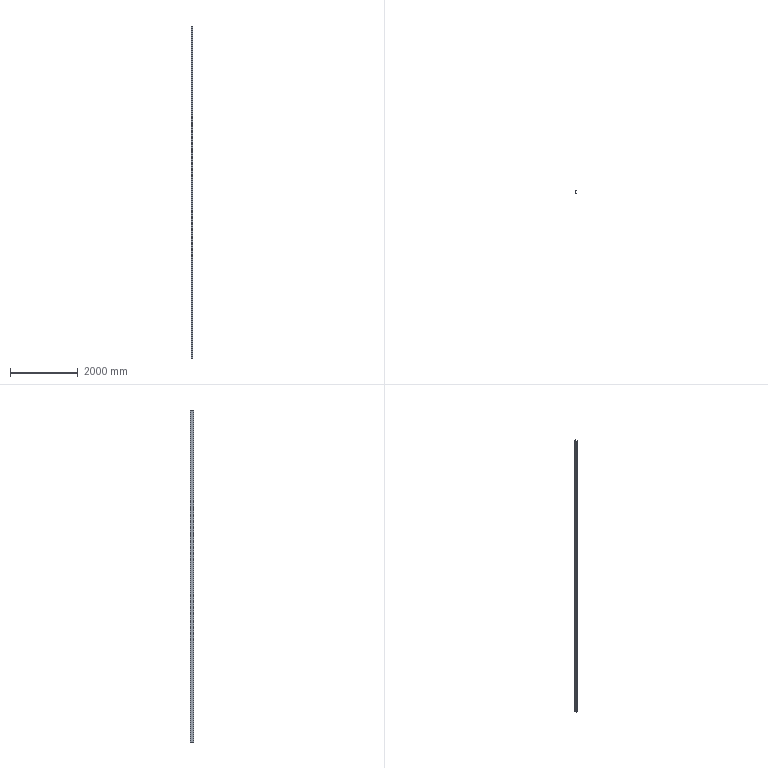Component | NX | CHUNSHUIJINCAO_CAOGANG | 1 solid | 10 faces | box 48 x 100 x 9820 mm | volume 12332938 mm3 | plane 10
STEP:
#1=CARTESIAN_POINT('',(0.,0.,0.));
#2=DIRECTION('',(0.,0.,1.));
#3=DIRECTION('',(1.,0.,0.));
#4=AXIS2_PLACEMENT_3D('',#1,#2,#3);
#5=CARTESIAN_POINT('',(2050.,9250.,9960.));
#6=VERTEX_POINT('',#5);
#7=CARTESIAN_POINT('',(2098.,9250.,9960.));
#8=VERTEX_POINT('',#7);
#9=CARTESIAN_POINT('',(2050.,9250.,9960.));
#10=DIRECTION('',(1.,0.,0.));
#11=VECTOR('',#10,1.);
#12=LINE('',#9,#11);
#13=CARTESIAN_POINT('',(2050.,9250.,140.));
#14=DIRECTION('',(0.,-1.,0.));
#15=DIRECTION('',(-1.,-0.,0.));
#16=AXIS2_PLACEMENT_3D('',#13,#14,#15);
#17=PLANE('',#16);
#18=CARTESIAN_POINT('',(0.,-9820.));
#19=DIRECTION('',(-1.,0.));
#20=VECTOR('',#19,1.);
#21=LINE('',#18,#20);
#22=(GEOMETRIC_REPRESENTATION_CONTEXT(2)PARAMETRIC_REPRESENTATION_CONTEXT()REPRESENTATION_CONTEXT('',''));
#23=DEFINITIONAL_REPRESENTATION('',(#21),#22);
#24=PCURVE('',#17,#23);
#25=CARTESIAN_POINT('',(2050.,9250.,9960.));
#26=DIRECTION('',(0.,0.,1.));
#27=DIRECTION('',(0.,-1.,0.));
#28=AXIS2_PLACEMENT_3D('',#25,#26,#27);
#29=PLANE('',#28);
#30=CARTESIAN_POINT('',(0.,0.));
#31=DIRECTION('',(-0.,1.));
#32=VECTOR('',#31,1.);
#33=LINE('',#30,#32);
#34=(GEOMETRIC_REPRESENTATION_CONTEXT(2)PARAMETRIC_REPRESENTATION_CONTEXT()REPRESENTATION_CONTEXT('',''));
#35=DEFINITIONAL_REPRESENTATION('',(#33),#34);
#36=PCURVE('',#29,#35);
#37=SURFACE_CURVE('',#12,(#24,#36),.PCURVE_S1.);
#38=EDGE_CURVE('',#6,#8,#37,.T.);
#39=ORIENTED_EDGE('',*,*,#38,.F.);
#40=CARTESIAN_POINT('',(2050.,9250.,140.));
#41=VERTEX_POINT('',#40);
#42=CARTESIAN_POINT('',(2050.,9250.,140.));
#43=DIRECTION('',(0.,0.,1.));
#44=VECTOR('',#43,1.);
#45=LINE('',#42,#44);
#46=CARTESIAN_POINT('',(0.,0.));
#47=DIRECTION('',(0.,-1.));
#48=VECTOR('',#47,1.);
#49=LINE('',#46,#48);
#50=(GEOMETRIC_REPRESENTATION_CONTEXT(2)PARAMETRIC_REPRESENTATION_CONTEXT()REPRESENTATION_CONTEXT('',''));
#51=DEFINITIONAL_REPRESENTATION('',(#49),#50);
#52=PCURVE('',#17,#51);
#53=CARTESIAN_POINT('',(2050.,9350.,140.));
#54=DIRECTION('',(-1.,0.,0.));
#55=DIRECTION('',(0.,0.,1.));
#56=AXIS2_PLACEMENT_3D('',#53,#54,#55);
#57=PLANE('',#56);
#58=CARTESIAN_POINT('',(0.,-100.));
#59=DIRECTION('',(1.,0.));
#60=VECTOR('',#59,1.);
#61=LINE('',#58,#60);
#62=(GEOMETRIC_REPRESENTATION_CONTEXT(2)PARAMETRIC_REPRESENTATION_CONTEXT()REPRESENTATION_CONTEXT('',''));
#63=DEFINITIONAL_REPRESENTATION('',(#61),#62);
#64=PCURVE('',#57,#63);
#65=SURFACE_CURVE('',#45,(#52,#64),.PCURVE_S1.);
#66=EDGE_CURVE('',#41,#6,#65,.T.);
#67=ORIENTED_EDGE('',*,*,#66,.F.);
#68=CARTESIAN_POINT('',(2098.,9250.,140.));
#69=VERTEX_POINT('',#68);
#70=CARTESIAN_POINT('',(2050.,9250.,140.));
#71=DIRECTION('',(1.,0.,0.));
#72=VECTOR('',#71,1.);
#73=LINE('',#70,#72);
#74=CARTESIAN_POINT('',(0.,0.));
#75=DIRECTION('',(-1.,0.));
#76=VECTOR('',#75,1.);
#77=LINE('',#74,#76);
#78=(GEOMETRIC_REPRESENTATION_CONTEXT(2)PARAMETRIC_REPRESENTATION_CONTEXT()REPRESENTATION_CONTEXT('',''));
#79=DEFINITIONAL_REPRESENTATION('',(#77),#78);
#80=PCURVE('',#17,#79);
#81=CARTESIAN_POINT('',(2050.,9250.,140.));
#82=DIRECTION('',(0.,0.,1.));
#83=DIRECTION('',(0.,-1.,0.));
#84=AXIS2_PLACEMENT_3D('',#81,#82,#83);
#85=PLANE('',#84);
#86=CARTESIAN_POINT('',(0.,0.));
#87=DIRECTION('',(-0.,1.));
#88=VECTOR('',#87,1.);
#89=LINE('',#86,#88);
#90=(GEOMETRIC_REPRESENTATION_CONTEXT(2)PARAMETRIC_REPRESENTATION_CONTEXT()REPRESENTATION_CONTEXT('',''));
#91=DEFINITIONAL_REPRESENTATION('',(#89),#90);
#92=PCURVE('',#85,#91);
#93=SURFACE_CURVE('',#73,(#80,#92),.PCURVE_S1.);
#94=EDGE_CURVE('',#41,#69,#93,.T.);
#95=ORIENTED_EDGE('',*,*,#94,.T.);
#96=CARTESIAN_POINT('',(2098.,9250.,140.));
#97=DIRECTION('',(0.,0.,1.));
#98=VECTOR('',#97,1.);
#99=LINE('',#96,#98);
#100=CARTESIAN_POINT('',(-48.,0.));
#101=DIRECTION('',(0.,-1.));
#102=VECTOR('',#101,1.);
#103=LINE('',#100,#102);
#104=(GEOMETRIC_REPRESENTATION_CONTEXT(2)PARAMETRIC_REPRESENTATION_CONTEXT()REPRESENTATION_CONTEXT('',''));
#105=DEFINITIONAL_REPRESENTATION('',(#103),#104);
#106=PCURVE('',#17,#105);
#107=CARTESIAN_POINT('',(2098.,9250.,140.));
#108=DIRECTION('',(1.,0.,0.));
#109=DIRECTION('',(0.,0.,-1.));
#110=AXIS2_PLACEMENT_3D('',#107,#108,#109);
#111=PLANE('',#110);
#112=CARTESIAN_POINT('',(0.,0.));
#113=DIRECTION('',(-1.,0.));
#114=VECTOR('',#113,1.);
#115=LINE('',#112,#114);
#116=(GEOMETRIC_REPRESENTATION_CONTEXT(2)PARAMETRIC_REPRESENTATION_CONTEXT()REPRESENTATION_CONTEXT('',''));
#117=DEFINITIONAL_REPRESENTATION('',(#115),#116);
#118=PCURVE('',#111,#117);
#119=SURFACE_CURVE('',#99,(#106,#118),.PCURVE_S1.);
#120=EDGE_CURVE('',#69,#8,#119,.T.);
#121=ORIENTED_EDGE('',*,*,#120,.T.);
#122=EDGE_LOOP('',(#39,#67,#95,#121));
#123=FACE_BOUND('',#122,.T.);
#124=ADVANCED_FACE('',(#123),#17,.T.);
#125=CARTESIAN_POINT('',(2098.,9258.5,9960.));
#126=VERTEX_POINT('',#125);
#127=CARTESIAN_POINT('',(2098.,9250.,9960.));
#128=DIRECTION('',(0.,1.,0.));
#129=VECTOR('',#128,1.);
#130=LINE('',#127,#129);
#131=CARTESIAN_POINT('',(-9820.,0.));
#132=DIRECTION('',(0.,1.));
#133=VECTOR('',#132,1.);
#134=LINE('',#131,#133);
#135=(GEOMETRIC_REPRESENTATION_CONTEXT(2)PARAMETRIC_REPRESENTATION_CONTEXT()REPRESENTATION_CONTEXT('',''));
#136=DEFINITIONAL_REPRESENTATION('',(#134),#135);
#137=PCURVE('',#111,#136);
#138=CARTESIAN_POINT('',(0.,48.));
#139=DIRECTION('',(-1.,0.));
#140=VECTOR('',#139,1.);
#141=LINE('',#138,#140);
#142=(GEOMETRIC_REPRESENTATION_CONTEXT(2)PARAMETRIC_REPRESENTATION_CONTEXT()REPRESENTATION_CONTEXT('',''));
#143=DEFINITIONAL_REPRESENTATION('',(#141),#142);
#144=PCURVE('',#29,#143);
#145=SURFACE_CURVE('',#130,(#137,#144),.PCURVE_S1.);
#146=EDGE_CURVE('',#8,#126,#145,.T.);
#147=ORIENTED_EDGE('',*,*,#146,.F.);
#148=ORIENTED_EDGE('',*,*,#120,.F.);
#149=CARTESIAN_POINT('',(2098.,9258.5,140.));
#150=VERTEX_POINT('',#149);
#151=CARTESIAN_POINT('',(2098.,9250.,140.));
#152=DIRECTION('',(0.,1.,0.));
#153=VECTOR('',#152,1.);
#154=LINE('',#151,#153);
#155=CARTESIAN_POINT('',(0.,0.));
#156=DIRECTION('',(0.,1.));
#157=VECTOR('',#156,1.);
#158=LINE('',#155,#157);
#159=(GEOMETRIC_REPRESENTATION_CONTEXT(2)PARAMETRIC_REPRESENTATION_CONTEXT()REPRESENTATION_CONTEXT('',''));
#160=DEFINITIONAL_REPRESENTATION('',(#158),#159);
#161=PCURVE('',#111,#160);
#162=CARTESIAN_POINT('',(0.,48.));
#163=DIRECTION('',(-1.,0.));
#164=VECTOR('',#163,1.);
#165=LINE('',#162,#164);
#166=(GEOMETRIC_REPRESENTATION_CONTEXT(2)PARAMETRIC_REPRESENTATION_CONTEXT()REPRESENTATION_CONTEXT('',''));
#167=DEFINITIONAL_REPRESENTATION('',(#165),#166);
#168=PCURVE('',#85,#167);
#169=SURFACE_CURVE('',#154,(#161,#168),.PCURVE_S1.);
#170=EDGE_CURVE('',#69,#150,#169,.T.);
#171=ORIENTED_EDGE('',*,*,#170,.T.);
#172=CARTESIAN_POINT('',(2098.,9258.5,140.));
#173=DIRECTION('',(0.,0.,1.));
#174=VECTOR('',#173,1.);
#175=LINE('',#172,#174);
#176=CARTESIAN_POINT('',(0.,8.5));
#177=DIRECTION('',(-1.,0.));
#178=VECTOR('',#177,1.);
#179=LINE('',#176,#178);
#180=(GEOMETRIC_REPRESENTATION_CONTEXT(2)PARAMETRIC_REPRESENTATION_CONTEXT()REPRESENTATION_CONTEXT('',''));
#181=DEFINITIONAL_REPRESENTATION('',(#179),#180);
#182=PCURVE('',#111,#181);
#183=CARTESIAN_POINT('',(2098.,9258.5,140.));
#184=DIRECTION('',(-0.,1.,0.));
#185=DIRECTION('',(1.,0.,0.));
#186=AXIS2_PLACEMENT_3D('',#183,#184,#185);
#187=PLANE('',#186);
#188=CARTESIAN_POINT('',(0.,0.));
#189=DIRECTION('',(0.,-1.));
#190=VECTOR('',#189,1.);
#191=LINE('',#188,#190);
#192=(GEOMETRIC_REPRESENTATION_CONTEXT(2)PARAMETRIC_REPRESENTATION_CONTEXT()REPRESENTATION_CONTEXT('',''));
#193=DEFINITIONAL_REPRESENTATION('',(#191),#192);
#194=PCURVE('',#187,#193);
#195=SURFACE_CURVE('',#175,(#182,#194),.PCURVE_S1.);
#196=EDGE_CURVE('',#150,#126,#195,.T.);
#197=ORIENTED_EDGE('',*,*,#196,.T.);
#198=EDGE_LOOP('',(#147,#148,#171,#197));
#199=FACE_BOUND('',#198,.T.);
#200=ADVANCED_FACE('',(#199),#111,.T.);
#201=CARTESIAN_POINT('',(2055.3,9258.5,9960.));
#202=VERTEX_POINT('',#201);
#203=CARTESIAN_POINT('',(2098.,9258.5,9960.));
#204=DIRECTION('',(-1.,-0.,0.));
#205=VECTOR('',#204,1.);
#206=LINE('',#203,#205);
#207=CARTESIAN_POINT('',(0.,-9820.));
#208=DIRECTION('',(-1.,0.));
#209=VECTOR('',#208,1.);
#210=LINE('',#207,#209);
#211=(GEOMETRIC_REPRESENTATION_CONTEXT(2)PARAMETRIC_REPRESENTATION_CONTEXT()REPRESENTATION_CONTEXT('',''));
#212=DEFINITIONAL_REPRESENTATION('',(#210),#211);
#213=PCURVE('',#187,#212);
#214=CARTESIAN_POINT('',(-8.5,48.));
#215=DIRECTION('',(0.,-1.));
#216=VECTOR('',#215,1.);
#217=LINE('',#214,#216);
#218=(GEOMETRIC_REPRESENTATION_CONTEXT(2)PARAMETRIC_REPRESENTATION_CONTEXT()REPRESENTATION_CONTEXT('',''));
#219=DEFINITIONAL_REPRESENTATION('',(#217),#218);
#220=PCURVE('',#29,#219);
#221=SURFACE_CURVE('',#206,(#213,#220),.PCURVE_S1.);
#222=EDGE_CURVE('',#126,#202,#221,.T.);
#223=ORIENTED_EDGE('',*,*,#222,.F.);
#224=ORIENTED_EDGE('',*,*,#196,.F.);
#225=CARTESIAN_POINT('',(2055.3,9258.5,140.));
#226=VERTEX_POINT('',#225);
#227=CARTESIAN_POINT('',(2098.,9258.5,140.));
#228=DIRECTION('',(-1.,-0.,0.));
#229=VECTOR('',#228,1.);
#230=LINE('',#227,#229);
#231=CARTESIAN_POINT('',(0.,0.));
#232=DIRECTION('',(-1.,0.));
#233=VECTOR('',#232,1.);
#234=LINE('',#231,#233);
#235=(GEOMETRIC_REPRESENTATION_CONTEXT(2)PARAMETRIC_REPRESENTATION_CONTEXT()REPRESENTATION_CONTEXT('',''));
#236=DEFINITIONAL_REPRESENTATION('',(#234),#235);
#237=PCURVE('',#187,#236);
#238=CARTESIAN_POINT('',(-8.5,48.));
#239=DIRECTION('',(0.,-1.));
#240=VECTOR('',#239,1.);
#241=LINE('',#238,#240);
#242=(GEOMETRIC_REPRESENTATION_CONTEXT(2)PARAMETRIC_REPRESENTATION_CONTEXT()REPRESENTATION_CONTEXT('',''));
#243=DEFINITIONAL_REPRESENTATION('',(#241),#242);
#244=PCURVE('',#85,#243);
#245=SURFACE_CURVE('',#230,(#237,#244),.PCURVE_S1.);
#246=EDGE_CURVE('',#150,#226,#245,.T.);
#247=ORIENTED_EDGE('',*,*,#246,.T.);
#248=CARTESIAN_POINT('',(2055.3,9258.5,140.));
#249=DIRECTION('',(0.,0.,1.));
#250=VECTOR('',#249,1.);
#251=LINE('',#248,#250);
#252=CARTESIAN_POINT('',(-42.7,0.));
#253=DIRECTION('',(0.,-1.));
#254=VECTOR('',#253,1.);
#255=LINE('',#252,#254);
#256=(GEOMETRIC_REPRESENTATION_CONTEXT(2)PARAMETRIC_REPRESENTATION_CONTEXT()REPRESENTATION_CONTEXT('',''));
#257=DEFINITIONAL_REPRESENTATION('',(#255),#256);
#258=PCURVE('',#187,#257);
#259=CARTESIAN_POINT('',(2055.3,9300.,140.));
#260=DIRECTION('',(1.,0.,0.));
#261=DIRECTION('',(0.,0.,-1.));
#262=AXIS2_PLACEMENT_3D('',#259,#260,#261);
#263=PLANE('',#262);
#264=CARTESIAN_POINT('',(0.,-41.5));
#265=DIRECTION('',(-1.,0.));
#266=VECTOR('',#265,1.);
#267=LINE('',#264,#266);
#268=(GEOMETRIC_REPRESENTATION_CONTEXT(2)PARAMETRIC_REPRESENTATION_CONTEXT()REPRESENTATION_CONTEXT('',''));
#269=DEFINITIONAL_REPRESENTATION('',(#267),#268);
#270=PCURVE('',#263,#269);
#271=SURFACE_CURVE('',#251,(#258,#270),.PCURVE_S1.);
#272=EDGE_CURVE('',#226,#202,#271,.T.);
#273=ORIENTED_EDGE('',*,*,#272,.T.);
#274=EDGE_LOOP('',(#223,#224,#247,#273));
#275=FACE_BOUND('',#274,.T.);
#276=ADVANCED_FACE('',(#275),#187,.T.);
#277=CARTESIAN_POINT('',(2055.3,9341.5,9960.));
#278=VERTEX_POINT('',#277);
#279=CARTESIAN_POINT('',(2055.3,9300.,9960.));
#280=DIRECTION('',(0.,1.,0.));
#281=VECTOR('',#280,1.);
#282=LINE('',#279,#281);
#283=CARTESIAN_POINT('',(-9820.,0.));
#284=DIRECTION('',(0.,1.));
#285=VECTOR('',#284,1.);
#286=LINE('',#283,#285);
#287=(GEOMETRIC_REPRESENTATION_CONTEXT(2)PARAMETRIC_REPRESENTATION_CONTEXT()REPRESENTATION_CONTEXT('',''));
#288=DEFINITIONAL_REPRESENTATION('',(#286),#287);
#289=PCURVE('',#263,#288);
#290=CARTESIAN_POINT('',(-50.,5.3));
#291=DIRECTION('',(-1.,0.));
#292=VECTOR('',#291,1.);
#293=LINE('',#290,#292);
#294=(GEOMETRIC_REPRESENTATION_CONTEXT(2)PARAMETRIC_REPRESENTATION_CONTEXT()REPRESENTATION_CONTEXT('',''));
#295=DEFINITIONAL_REPRESENTATION('',(#293),#294);
#296=PCURVE('',#29,#295);
#297=SURFACE_CURVE('',#282,(#289,#296),.PCURVE_S1.);
#298=EDGE_CURVE('',#202,#278,#297,.T.);
#299=ORIENTED_EDGE('',*,*,#298,.F.);
#300=ORIENTED_EDGE('',*,*,#272,.F.);
#301=CARTESIAN_POINT('',(2055.3,9341.5,140.));
#302=VERTEX_POINT('',#301);
#303=CARTESIAN_POINT('',(2055.3,9258.5,140.));
#304=DIRECTION('',(-0.,1.,0.));
#305=VECTOR('',#304,1.);
#306=LINE('',#303,#305);
#307=CARTESIAN_POINT('',(0.,-41.5));
#308=DIRECTION('',(0.,1.));
#309=VECTOR('',#308,1.);
#310=LINE('',#307,#309);
#311=(GEOMETRIC_REPRESENTATION_CONTEXT(2)PARAMETRIC_REPRESENTATION_CONTEXT()REPRESENTATION_CONTEXT('',''));
#312=DEFINITIONAL_REPRESENTATION('',(#310),#311);
#313=PCURVE('',#263,#312);
#314=CARTESIAN_POINT('',(-8.5,5.3));
#315=DIRECTION('',(-1.,-0.));
#316=VECTOR('',#315,1.);
#317=LINE('',#314,#316);
#318=(GEOMETRIC_REPRESENTATION_CONTEXT(2)PARAMETRIC_REPRESENTATION_CONTEXT()REPRESENTATION_CONTEXT('',''));
#319=DEFINITIONAL_REPRESENTATION('',(#317),#318);
#320=PCURVE('',#85,#319);
#321=SURFACE_CURVE('',#306,(#313,#320),.PCURVE_S1.);
#322=EDGE_CURVE('',#226,#302,#321,.T.);
#323=ORIENTED_EDGE('',*,*,#322,.T.);
#324=CARTESIAN_POINT('',(2055.3,9341.5,140.));
#325=DIRECTION('',(0.,0.,1.));
#326=VECTOR('',#325,1.);
#327=LINE('',#324,#326);
#328=CARTESIAN_POINT('',(0.,41.5));
#329=DIRECTION('',(-1.,0.));
#330=VECTOR('',#329,1.);
#331=LINE('',#328,#330);
#332=(GEOMETRIC_REPRESENTATION_CONTEXT(2)PARAMETRIC_REPRESENTATION_CONTEXT()REPRESENTATION_CONTEXT('',''));
#333=DEFINITIONAL_REPRESENTATION('',(#331),#332);
#334=PCURVE('',#263,#333);
#335=CARTESIAN_POINT('',(2055.3,9341.5,140.));
#336=DIRECTION('',(0.,-1.,0.));
#337=DIRECTION('',(-1.,-0.,0.));
#338=AXIS2_PLACEMENT_3D('',#335,#336,#337);
#339=PLANE('',#338);
#340=CARTESIAN_POINT('',(0.,0.));
#341=DIRECTION('',(0.,-1.));
#342=VECTOR('',#341,1.);
#343=LINE('',#340,#342);
#344=(GEOMETRIC_REPRESENTATION_CONTEXT(2)PARAMETRIC_REPRESENTATION_CONTEXT()REPRESENTATION_CONTEXT('',''));
#345=DEFINITIONAL_REPRESENTATION('',(#343),#344);
#346=PCURVE('',#339,#345);
#347=SURFACE_CURVE('',#327,(#334,#346),.PCURVE_S1.);
#348=EDGE_CURVE('',#302,#278,#347,.T.);
#349=ORIENTED_EDGE('',*,*,#348,.T.);
#350=EDGE_LOOP('',(#299,#300,#323,#349));
#351=FACE_BOUND('',#350,.T.);
#352=ADVANCED_FACE('',(#351),#263,.T.);
#353=CARTESIAN_POINT('',(2098.,9341.5,9960.));
#354=VERTEX_POINT('',#353);
#355=CARTESIAN_POINT('',(2055.3,9341.5,9960.));
#356=DIRECTION('',(1.,0.,0.));
#357=VECTOR('',#356,1.);
#358=LINE('',#355,#357);
#359=CARTESIAN_POINT('',(0.,-9820.));
#360=DIRECTION('',(-1.,0.));
#361=VECTOR('',#360,1.);
#362=LINE('',#359,#361);
#363=(GEOMETRIC_REPRESENTATION_CONTEXT(2)PARAMETRIC_REPRESENTATION_CONTEXT()REPRESENTATION_CONTEXT('',''));
#364=DEFINITIONAL_REPRESENTATION('',(#362),#363);
#365=PCURVE('',#339,#364);
#366=CARTESIAN_POINT('',(-91.5,5.3));
#367=DIRECTION('',(-0.,1.));
#368=VECTOR('',#367,1.);
#369=LINE('',#366,#368);
#370=(GEOMETRIC_REPRESENTATION_CONTEXT(2)PARAMETRIC_REPRESENTATION_CONTEXT()REPRESENTATION_CONTEXT('',''));
#371=DEFINITIONAL_REPRESENTATION('',(#369),#370);
#372=PCURVE('',#29,#371);
#373=SURFACE_CURVE('',#358,(#365,#372),.PCURVE_S1.);
#374=EDGE_CURVE('',#278,#354,#373,.T.);
#375=ORIENTED_EDGE('',*,*,#374,.F.);
#376=ORIENTED_EDGE('',*,*,#348,.F.);
#377=CARTESIAN_POINT('',(2098.,9341.5,140.));
#378=VERTEX_POINT('',#377);
#379=CARTESIAN_POINT('',(2055.3,9341.5,140.));
#380=DIRECTION('',(1.,0.,0.));
#381=VECTOR('',#380,1.);
#382=LINE('',#379,#381);
#383=CARTESIAN_POINT('',(0.,0.));
#384=DIRECTION('',(-1.,0.));
#385=VECTOR('',#384,1.);
#386=LINE('',#383,#385);
#387=(GEOMETRIC_REPRESENTATION_CONTEXT(2)PARAMETRIC_REPRESENTATION_CONTEXT()REPRESENTATION_CONTEXT('',''));
#388=DEFINITIONAL_REPRESENTATION('',(#386),#387);
#389=PCURVE('',#339,#388);
#390=CARTESIAN_POINT('',(-91.5,5.3));
#391=DIRECTION('',(-0.,1.));
#392=VECTOR('',#391,1.);
#393=LINE('',#390,#392);
#394=(GEOMETRIC_REPRESENTATION_CONTEXT(2)PARAMETRIC_REPRESENTATION_CONTEXT()REPRESENTATION_CONTEXT('',''));
#395=DEFINITIONAL_REPRESENTATION('',(#393),#394);
#396=PCURVE('',#85,#395);
#397=SURFACE_CURVE('',#382,(#389,#396),.PCURVE_S1.);
#398=EDGE_CURVE('',#302,#378,#397,.T.);
#399=ORIENTED_EDGE('',*,*,#398,.T.);
#400=CARTESIAN_POINT('',(2098.,9341.5,140.));
#401=DIRECTION('',(0.,0.,1.));
#402=VECTOR('',#401,1.);
#403=LINE('',#400,#402);
#404=CARTESIAN_POINT('',(-42.7,0.));
#405=DIRECTION('',(0.,-1.));
#406=VECTOR('',#405,1.);
#407=LINE('',#404,#406);
#408=(GEOMETRIC_REPRESENTATION_CONTEXT(2)PARAMETRIC_REPRESENTATION_CONTEXT()REPRESENTATION_CONTEXT('',''));
#409=DEFINITIONAL_REPRESENTATION('',(#407),#408);
#410=PCURVE('',#339,#409);
#411=CARTESIAN_POINT('',(2098.,9341.5,140.));
#412=DIRECTION('',(1.,0.,0.));
#413=DIRECTION('',(0.,-1.,0.));
#414=AXIS2_PLACEMENT_3D('',#411,#412,#413);
#415=PLANE('',#414);
#416=CARTESIAN_POINT('',(0.,0.));
#417=DIRECTION('',(0.,-1.));
#418=VECTOR('',#417,1.);
#419=LINE('',#416,#418);
#420=(GEOMETRIC_REPRESENTATION_CONTEXT(2)PARAMETRIC_REPRESENTATION_CONTEXT()REPRESENTATION_CONTEXT('',''));
#421=DEFINITIONAL_REPRESENTATION('',(#419),#420);
#422=PCURVE('',#415,#421);
#423=SURFACE_CURVE('',#403,(#410,#422),.PCURVE_S1.);
#424=EDGE_CURVE('',#378,#354,#423,.T.);
#425=ORIENTED_EDGE('',*,*,#424,.T.);
#426=EDGE_LOOP('',(#375,#376,#399,#425));
#427=FACE_BOUND('',#426,.T.);
#428=ADVANCED_FACE('',(#427),#339,.T.);
#429=CARTESIAN_POINT('',(2098.,9350.,9960.));
#430=VERTEX_POINT('',#429);
#431=CARTESIAN_POINT('',(2098.,9341.5,9960.));
#432=DIRECTION('',(-0.,1.,0.));
#433=VECTOR('',#432,1.);
#434=LINE('',#431,#433);
#435=CARTESIAN_POINT('',(0.,-9820.));
#436=DIRECTION('',(-1.,0.));
#437=VECTOR('',#436,1.);
#438=LINE('',#435,#437);
#439=(GEOMETRIC_REPRESENTATION_CONTEXT(2)PARAMETRIC_REPRESENTATION_CONTEXT()REPRESENTATION_CONTEXT('',''));
#440=DEFINITIONAL_REPRESENTATION('',(#438),#439);
#441=PCURVE('',#415,#440);
#442=CARTESIAN_POINT('',(-91.5,48.));
#443=DIRECTION('',(-1.,-0.));
#444=VECTOR('',#443,1.);
#445=LINE('',#442,#444);
#446=(GEOMETRIC_REPRESENTATION_CONTEXT(2)PARAMETRIC_REPRESENTATION_CONTEXT()REPRESENTATION_CONTEXT('',''));
#447=DEFINITIONAL_REPRESENTATION('',(#445),#446);
#448=PCURVE('',#29,#447);
#449=SURFACE_CURVE('',#434,(#441,#448),.PCURVE_S1.);
#450=EDGE_CURVE('',#354,#430,#449,.T.);
#451=ORIENTED_EDGE('',*,*,#450,.F.);
#452=ORIENTED_EDGE('',*,*,#424,.F.);
#453=CARTESIAN_POINT('',(2098.,9350.,140.));
#454=VERTEX_POINT('',#453);
#455=CARTESIAN_POINT('',(2098.,9341.5,140.));
#456=DIRECTION('',(-0.,1.,0.));
#457=VECTOR('',#456,1.);
#458=LINE('',#455,#457);
#459=CARTESIAN_POINT('',(0.,0.));
#460=DIRECTION('',(-1.,0.));
#461=VECTOR('',#460,1.);
#462=LINE('',#459,#461);
#463=(GEOMETRIC_REPRESENTATION_CONTEXT(2)PARAMETRIC_REPRESENTATION_CONTEXT()REPRESENTATION_CONTEXT('',''));
#464=DEFINITIONAL_REPRESENTATION('',(#462),#463);
#465=PCURVE('',#415,#464);
#466=CARTESIAN_POINT('',(-91.5,48.));
#467=DIRECTION('',(-1.,-0.));
#468=VECTOR('',#467,1.);
#469=LINE('',#466,#468);
#470=(GEOMETRIC_REPRESENTATION_CONTEXT(2)PARAMETRIC_REPRESENTATION_CONTEXT()REPRESENTATION_CONTEXT('',''));
#471=DEFINITIONAL_REPRESENTATION('',(#469),#470);
#472=PCURVE('',#85,#471);
#473=SURFACE_CURVE('',#458,(#465,#472),.PCURVE_S1.);
#474=EDGE_CURVE('',#378,#454,#473,.T.);
#475=ORIENTED_EDGE('',*,*,#474,.T.);
#476=CARTESIAN_POINT('',(2098.,9350.,140.));
#477=DIRECTION('',(0.,0.,1.));
#478=VECTOR('',#477,1.);
#479=LINE('',#476,#478);
#480=CARTESIAN_POINT('',(-8.5,0.));
#481=DIRECTION('',(0.,-1.));
#482=VECTOR('',#481,1.);
#483=LINE('',#480,#482);
#484=(GEOMETRIC_REPRESENTATION_CONTEXT(2)PARAMETRIC_REPRESENTATION_CONTEXT()REPRESENTATION_CONTEXT('',''));
#485=DEFINITIONAL_REPRESENTATION('',(#483),#484);
#486=PCURVE('',#415,#485);
#487=CARTESIAN_POINT('',(2098.,9350.,140.));
#488=DIRECTION('',(-0.,1.,0.));
#489=DIRECTION('',(1.,0.,0.));
#490=AXIS2_PLACEMENT_3D('',#487,#488,#489);
#491=PLANE('',#490);
#492=CARTESIAN_POINT('',(0.,0.));
#493=DIRECTION('',(0.,-1.));
#494=VECTOR('',#493,1.);
#495=LINE('',#492,#494);
#496=(GEOMETRIC_REPRESENTATION_CONTEXT(2)PARAMETRIC_REPRESENTATION_CONTEXT()REPRESENTATION_CONTEXT('',''));
#497=DEFINITIONAL_REPRESENTATION('',(#495),#496);
#498=PCURVE('',#491,#497);
#499=SURFACE_CURVE('',#479,(#486,#498),.PCURVE_S1.);
#500=EDGE_CURVE('',#454,#430,#499,.T.);
#501=ORIENTED_EDGE('',*,*,#500,.T.);
#502=EDGE_LOOP('',(#451,#452,#475,#501));
#503=FACE_BOUND('',#502,.T.);
#504=ADVANCED_FACE('',(#503),#415,.T.);
#505=CARTESIAN_POINT('',(2050.,9350.,9960.));
#506=VERTEX_POINT('',#505);
#507=CARTESIAN_POINT('',(2098.,9350.,9960.));
#508=DIRECTION('',(-1.,-0.,0.));
#509=VECTOR('',#508,1.);
#510=LINE('',#507,#509);
#511=CARTESIAN_POINT('',(0.,-9820.));
#512=DIRECTION('',(-1.,0.));
#513=VECTOR('',#512,1.);
#514=LINE('',#511,#513);
#515=(GEOMETRIC_REPRESENTATION_CONTEXT(2)PARAMETRIC_REPRESENTATION_CONTEXT()REPRESENTATION_CONTEXT('',''));
#516=DEFINITIONAL_REPRESENTATION('',(#514),#515);
#517=PCURVE('',#491,#516);
#518=CARTESIAN_POINT('',(-100.,48.));
#519=DIRECTION('',(0.,-1.));
#520=VECTOR('',#519,1.);
#521=LINE('',#518,#520);
#522=(GEOMETRIC_REPRESENTATION_CONTEXT(2)PARAMETRIC_REPRESENTATION_CONTEXT()REPRESENTATION_CONTEXT('',''));
#523=DEFINITIONAL_REPRESENTATION('',(#521),#522);
#524=PCURVE('',#29,#523);
#525=SURFACE_CURVE('',#510,(#517,#524),.PCURVE_S1.);
#526=EDGE_CURVE('',#430,#506,#525,.T.);
#527=ORIENTED_EDGE('',*,*,#526,.F.);
#528=ORIENTED_EDGE('',*,*,#500,.F.);
#529=CARTESIAN_POINT('',(2050.,9350.,140.));
#530=VERTEX_POINT('',#529);
#531=CARTESIAN_POINT('',(2098.,9350.,140.));
#532=DIRECTION('',(-1.,-0.,0.));
#533=VECTOR('',#532,1.);
#534=LINE('',#531,#533);
#535=CARTESIAN_POINT('',(0.,0.));
#536=DIRECTION('',(-1.,0.));
#537=VECTOR('',#536,1.);
#538=LINE('',#535,#537);
#539=(GEOMETRIC_REPRESENTATION_CONTEXT(2)PARAMETRIC_REPRESENTATION_CONTEXT()REPRESENTATION_CONTEXT('',''));
#540=DEFINITIONAL_REPRESENTATION('',(#538),#539);
#541=PCURVE('',#491,#540);
#542=CARTESIAN_POINT('',(-100.,48.));
#543=DIRECTION('',(0.,-1.));
#544=VECTOR('',#543,1.);
#545=LINE('',#542,#544);
#546=(GEOMETRIC_REPRESENTATION_CONTEXT(2)PARAMETRIC_REPRESENTATION_CONTEXT()REPRESENTATION_CONTEXT('',''));
#547=DEFINITIONAL_REPRESENTATION('',(#545),#546);
#548=PCURVE('',#85,#547);
#549=SURFACE_CURVE('',#534,(#541,#548),.PCURVE_S1.);
#550=EDGE_CURVE('',#454,#530,#549,.T.);
#551=ORIENTED_EDGE('',*,*,#550,.T.);
#552=CARTESIAN_POINT('',(2050.,9350.,140.));
#553=DIRECTION('',(0.,0.,1.));
#554=VECTOR('',#553,1.);
#555=LINE('',#552,#554);
#556=CARTESIAN_POINT('',(-48.,0.));
#557=DIRECTION('',(0.,-1.));
#558=VECTOR('',#557,1.);
#559=LINE('',#556,#558);
#560=(GEOMETRIC_REPRESENTATION_CONTEXT(2)PARAMETRIC_REPRESENTATION_CONTEXT()REPRESENTATION_CONTEXT('',''));
#561=DEFINITIONAL_REPRESENTATION('',(#559),#560);
#562=PCURVE('',#491,#561);
#563=CARTESIAN_POINT('',(0.,0.));
#564=DIRECTION('',(1.,0.));
#565=VECTOR('',#564,1.);
#566=LINE('',#563,#565);
#567=(GEOMETRIC_REPRESENTATION_CONTEXT(2)PARAMETRIC_REPRESENTATION_CONTEXT()REPRESENTATION_CONTEXT('',''));
#568=DEFINITIONAL_REPRESENTATION('',(#566),#567);
#569=PCURVE('',#57,#568);
#570=SURFACE_CURVE('',#555,(#562,#569),.PCURVE_S1.);
#571=EDGE_CURVE('',#530,#506,#570,.T.);
#572=ORIENTED_EDGE('',*,*,#571,.T.);
#573=EDGE_LOOP('',(#527,#528,#551,#572));
#574=FACE_BOUND('',#573,.T.);
#575=ADVANCED_FACE('',(#574),#491,.T.);
#576=CARTESIAN_POINT('',(2050.,9350.,9960.));
#577=DIRECTION('',(0.,-1.,0.));
#578=VECTOR('',#577,1.);
#579=LINE('',#576,#578);
#580=CARTESIAN_POINT('',(9820.,0.));
#581=DIRECTION('',(0.,-1.));
#582=VECTOR('',#581,1.);
#583=LINE('',#580,#582);
#584=(GEOMETRIC_REPRESENTATION_CONTEXT(2)PARAMETRIC_REPRESENTATION_CONTEXT()REPRESENTATION_CONTEXT('',''));
#585=DEFINITIONAL_REPRESENTATION('',(#583),#584);
#586=PCURVE('',#57,#585);
#587=CARTESIAN_POINT('',(-100.,0.));
#588=DIRECTION('',(1.,0.));
#589=VECTOR('',#588,1.);
#590=LINE('',#587,#589);
#591=(GEOMETRIC_REPRESENTATION_CONTEXT(2)PARAMETRIC_REPRESENTATION_CONTEXT()REPRESENTATION_CONTEXT('',''));
#592=DEFINITIONAL_REPRESENTATION('',(#590),#591);
#593=PCURVE('',#29,#592);
#594=SURFACE_CURVE('',#579,(#586,#593),.PCURVE_S1.);
#595=EDGE_CURVE('',#506,#6,#594,.T.);
#596=ORIENTED_EDGE('',*,*,#595,.F.);
#597=ORIENTED_EDGE('',*,*,#571,.F.);
#598=CARTESIAN_POINT('',(2050.,9350.,140.));
#599=DIRECTION('',(0.,-1.,0.));
#600=VECTOR('',#599,1.);
#601=LINE('',#598,#600);
#602=CARTESIAN_POINT('',(0.,0.));
#603=DIRECTION('',(0.,-1.));
#604=VECTOR('',#603,1.);
#605=LINE('',#602,#604);
#606=(GEOMETRIC_REPRESENTATION_CONTEXT(2)PARAMETRIC_REPRESENTATION_CONTEXT()REPRESENTATION_CONTEXT('',''));
#607=DEFINITIONAL_REPRESENTATION('',(#605),#606);
#608=PCURVE('',#57,#607);
#609=CARTESIAN_POINT('',(-100.,0.));
#610=DIRECTION('',(1.,0.));
#611=VECTOR('',#610,1.);
#612=LINE('',#609,#611);
#613=(GEOMETRIC_REPRESENTATION_CONTEXT(2)PARAMETRIC_REPRESENTATION_CONTEXT()REPRESENTATION_CONTEXT('',''));
#614=DEFINITIONAL_REPRESENTATION('',(#612),#613);
#615=PCURVE('',#85,#614);
#616=SURFACE_CURVE('',#601,(#608,#615),.PCURVE_S1.);
#617=EDGE_CURVE('',#530,#41,#616,.T.);
#618=ORIENTED_EDGE('',*,*,#617,.T.);
#619=ORIENTED_EDGE('',*,*,#66,.T.);
#620=EDGE_LOOP('',(#596,#597,#618,#619));
#621=FACE_BOUND('',#620,.T.);
#622=ADVANCED_FACE('',(#621),#57,.T.);
#623=ORIENTED_EDGE('',*,*,#94,.F.);
#624=ORIENTED_EDGE('',*,*,#617,.F.);
#625=ORIENTED_EDGE('',*,*,#550,.F.);
#626=ORIENTED_EDGE('',*,*,#474,.F.);
#627=ORIENTED_EDGE('',*,*,#398,.F.);
#628=ORIENTED_EDGE('',*,*,#322,.F.);
#629=ORIENTED_EDGE('',*,*,#246,.F.);
#630=ORIENTED_EDGE('',*,*,#170,.F.);
#631=EDGE_LOOP('',(#623,#624,#625,#626,#627,#628,#629,#630));
#632=FACE_BOUND('',#631,.T.);
#633=ADVANCED_FACE('',(#632),#85,.F.);
#634=ORIENTED_EDGE('',*,*,#38,.T.);
#635=ORIENTED_EDGE('',*,*,#146,.T.);
#636=ORIENTED_EDGE('',*,*,#222,.T.);
#637=ORIENTED_EDGE('',*,*,#298,.T.);
#638=ORIENTED_EDGE('',*,*,#374,.T.);
#639=ORIENTED_EDGE('',*,*,#450,.T.);
#640=ORIENTED_EDGE('',*,*,#526,.T.);
#641=ORIENTED_EDGE('',*,*,#595,.T.);
#642=EDGE_LOOP('',(#634,#635,#636,#637,#638,#639,#640,#641));
#643=FACE_BOUND('',#642,.T.);
#644=ADVANCED_FACE('',(#643),#29,.T.);
#645=CLOSED_SHELL('',(#124,#200,#276,#352,#428,#504,#575,#622,#633,#644));
#646=MANIFOLD_SOLID_BREP('',#645);
#647=(LENGTH_UNIT()NAMED_UNIT(*)SI_UNIT(.MILLI.,.METRE.));
#648=UNCERTAINTY_MEASURE_WITH_UNIT(LENGTH_MEASURE(0.0000001),#647,'','');
#649=(NAMED_UNIT(*)PLANE_ANGLE_UNIT()SI_UNIT($,.RADIAN.));
#650=(NAMED_UNIT(*)SI_UNIT($,.STERADIAN.)SOLID_ANGLE_UNIT());
#651=(GEOMETRIC_REPRESENTATION_CONTEXT(3)GLOBAL_UNCERTAINTY_ASSIGNED_CONTEXT((#648))GLOBAL_UNIT_ASSIGNED_CONTEXT((#647,#649,#650))REPRESENTATION_CONTEXT('',''));
#652=ADVANCED_BREP_SHAPE_REPRESENTATION('',(#4,#646),#651);